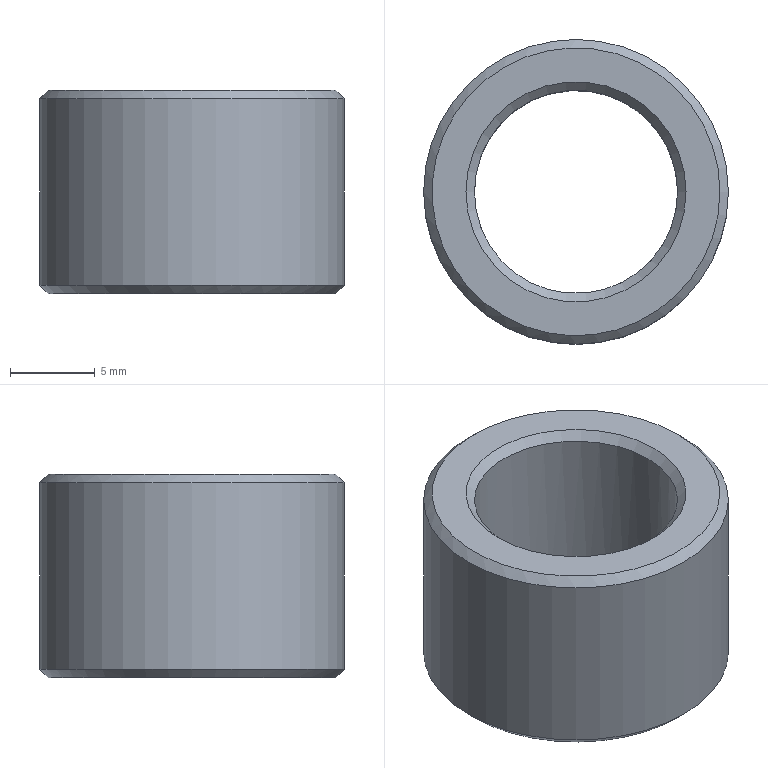Component | NX | BUSHING | 1 solid | 8 faces | box 18 x 18 x 12 mm | volume 1673 mm3 | cone 4 | plane 2 | cylinder 2 | commonest cylinder face diameters 18 x1 12 x1
STEP:
#1=CARTESIAN_POINT('',(0.,0.,0.));
#2=DIRECTION('',(0.,0.,1.));
#3=DIRECTION('',(1.,0.,0.));
#4=AXIS2_PLACEMENT_3D('',#1,#2,#3);
#5=CARTESIAN_POINT('',(17.728,-17.527,-161.719));
#6=VERTEX_POINT('',#5);
#7=CARTESIAN_POINT('',(11.228,-17.527,-161.719));
#8=DIRECTION('',(0.,0.,-1.));
#9=DIRECTION('',(1.,0.,0.));
#10=AXIS2_PLACEMENT_3D('',#7,#8,#9);
#11=CIRCLE('',#10,6.5);
#12=CARTESIAN_POINT('',(11.228,-17.527,-161.719));
#13=DIRECTION('',(0.,0.,1.));
#14=DIRECTION('',(1.,0.,0.));
#15=AXIS2_PLACEMENT_3D('',#12,#13,#14);
#16=PLANE('',#15);
#17=CARTESIAN_POINT('',(6.5,0.));
#18=CARTESIAN_POINT('',(6.5,-11.258));
#19=CARTESIAN_POINT('',(-3.25,-5.629));
#20=CARTESIAN_POINT('',(-13.,-0.));
#21=CARTESIAN_POINT('',(-3.25,5.629));
#22=CARTESIAN_POINT('',(6.5,11.258));
#23=CARTESIAN_POINT('',(6.5,0.));
#24=(BOUNDED_CURVE()B_SPLINE_CURVE(2,(#17,#18,#19,#20,#21,#22,#23),.UNSPECIFIED.,.T.,.F.)B_SPLINE_CURVE_WITH_KNOTS((1,2,2,2,2,1),(-2.094,0.,2.094,4.189,6.283,8.378),.UNSPECIFIED.)CURVE()GEOMETRIC_REPRESENTATION_ITEM()RATIONAL_B_SPLINE_CURVE((1.,0.5,1.,0.5,1.,0.5,1.))REPRESENTATION_ITEM(''));
#25=(GEOMETRIC_REPRESENTATION_CONTEXT(2)PARAMETRIC_REPRESENTATION_CONTEXT()REPRESENTATION_CONTEXT('',''));
#26=DEFINITIONAL_REPRESENTATION('',(#24),#25);
#27=PCURVE('',#16,#26);
#28=CARTESIAN_POINT('',(11.228,-17.527,-161.719));
#29=DIRECTION('',(0.,0.,1.));
#30=DIRECTION('',(1.,0.,0.));
#31=AXIS2_PLACEMENT_3D('',#28,#29,#30);
#32=CONICAL_SURFACE('',#31,6.5,0.7854);
#33=CARTESIAN_POINT('',(6.283,0.));
#34=DIRECTION('',(-1.,0.));
#35=VECTOR('',#34,1.);
#36=LINE('',#33,#35);
#37=(GEOMETRIC_REPRESENTATION_CONTEXT(2)PARAMETRIC_REPRESENTATION_CONTEXT()REPRESENTATION_CONTEXT('',''));
#38=DEFINITIONAL_REPRESENTATION('',(#36),#37);
#39=PCURVE('',#32,#38);
#40=SURFACE_CURVE('',#11,(#27,#39),.PCURVE_S1.);
#41=EDGE_CURVE('',#6,#6,#40,.T.);
#42=ORIENTED_EDGE('',*,*,#41,.T.);
#43=EDGE_LOOP('',(#42));
#44=FACE_BOUND('',#43,.T.);
#45=CARTESIAN_POINT('',(19.728,-17.527,-161.719));
#46=VERTEX_POINT('',#45);
#47=CARTESIAN_POINT('',(11.228,-17.527,-161.719));
#48=DIRECTION('',(0.,0.,1.));
#49=DIRECTION('',(1.,0.,0.));
#50=AXIS2_PLACEMENT_3D('',#47,#48,#49);
#51=CIRCLE('',#50,8.5);
#52=CARTESIAN_POINT('',(0.,0.));
#53=DIRECTION('',(1.,0.));
#54=AXIS2_PLACEMENT_2D('',#52,#53);
#55=CIRCLE('',#54,8.5);
#56=(GEOMETRIC_REPRESENTATION_CONTEXT(2)PARAMETRIC_REPRESENTATION_CONTEXT()REPRESENTATION_CONTEXT('',''));
#57=DEFINITIONAL_REPRESENTATION('',(#55),#56);
#58=PCURVE('',#16,#57);
#59=CARTESIAN_POINT('',(11.228,-17.527,-162.219));
#60=DIRECTION('',(0.,0.,-1.));
#61=DIRECTION('',(-1.,0.,0.));
#62=AXIS2_PLACEMENT_3D('',#59,#60,#61);
#63=CONICAL_SURFACE('',#62,9.,0.7854);
#64=CARTESIAN_POINT('',(9.425,-0.5));
#65=DIRECTION('',(-1.,0.));
#66=VECTOR('',#65,1.);
#67=LINE('',#64,#66);
#68=(GEOMETRIC_REPRESENTATION_CONTEXT(2)PARAMETRIC_REPRESENTATION_CONTEXT()REPRESENTATION_CONTEXT('',''));
#69=DEFINITIONAL_REPRESENTATION('',(#67),#68);
#70=PCURVE('',#63,#69);
#71=SURFACE_CURVE('',#51,(#58,#70),.PCURVE_S1.);
#72=EDGE_CURVE('',#46,#46,#71,.T.);
#73=ORIENTED_EDGE('',*,*,#72,.T.);
#74=EDGE_LOOP('',(#73));
#75=FACE_BOUND('',#74,.T.);
#76=ADVANCED_FACE('',(#44,#75),#16,.T.);
#77=CARTESIAN_POINT('',(4.728,-17.527,-173.719));
#78=VERTEX_POINT('',#77);
#79=CARTESIAN_POINT('',(11.228,-17.527,-173.719));
#80=DIRECTION('',(0.,0.,1.));
#81=DIRECTION('',(-1.,0.,0.));
#82=AXIS2_PLACEMENT_3D('',#79,#80,#81);
#83=CIRCLE('',#82,6.5);
#84=CARTESIAN_POINT('',(11.228,-17.527,-173.719));
#85=DIRECTION('',(0.,0.,-1.));
#86=DIRECTION('',(-1.,0.,0.));
#87=AXIS2_PLACEMENT_3D('',#84,#85,#86);
#88=PLANE('',#87);
#89=CARTESIAN_POINT('',(6.5,0.));
#90=CARTESIAN_POINT('',(6.5,-11.258));
#91=CARTESIAN_POINT('',(-3.25,-5.629));
#92=CARTESIAN_POINT('',(-13.,-0.));
#93=CARTESIAN_POINT('',(-3.25,5.629));
#94=CARTESIAN_POINT('',(6.5,11.258));
#95=CARTESIAN_POINT('',(6.5,0.));
#96=(BOUNDED_CURVE()B_SPLINE_CURVE(2,(#89,#90,#91,#92,#93,#94,#95),.UNSPECIFIED.,.T.,.F.)B_SPLINE_CURVE_WITH_KNOTS((1,2,2,2,2,1),(-2.094,0.,2.094,4.189,6.283,8.378),.UNSPECIFIED.)CURVE()GEOMETRIC_REPRESENTATION_ITEM()RATIONAL_B_SPLINE_CURVE((1.,0.5,1.,0.5,1.,0.5,1.))REPRESENTATION_ITEM(''));
#97=(GEOMETRIC_REPRESENTATION_CONTEXT(2)PARAMETRIC_REPRESENTATION_CONTEXT()REPRESENTATION_CONTEXT('',''));
#98=DEFINITIONAL_REPRESENTATION('',(#96),#97);
#99=PCURVE('',#88,#98);
#100=CARTESIAN_POINT('',(11.228,-17.527,-173.219));
#101=DIRECTION('',(0.,0.,-1.));
#102=DIRECTION('',(-1.,0.,0.));
#103=AXIS2_PLACEMENT_3D('',#100,#101,#102);
#104=CONICAL_SURFACE('',#103,6.,0.7854);
#105=CARTESIAN_POINT('',(6.283,0.5));
#106=DIRECTION('',(-1.,0.));
#107=VECTOR('',#106,1.);
#108=LINE('',#105,#107);
#109=(GEOMETRIC_REPRESENTATION_CONTEXT(2)PARAMETRIC_REPRESENTATION_CONTEXT()REPRESENTATION_CONTEXT('',''));
#110=DEFINITIONAL_REPRESENTATION('',(#108),#109);
#111=PCURVE('',#104,#110);
#112=SURFACE_CURVE('',#83,(#99,#111),.PCURVE_S1.);
#113=EDGE_CURVE('',#78,#78,#112,.T.);
#114=ORIENTED_EDGE('',*,*,#113,.T.);
#115=EDGE_LOOP('',(#114));
#116=FACE_BOUND('',#115,.T.);
#117=CARTESIAN_POINT('',(2.728,-17.527,-173.719));
#118=VERTEX_POINT('',#117);
#119=CARTESIAN_POINT('',(11.228,-17.527,-173.719));
#120=DIRECTION('',(0.,0.,-1.));
#121=DIRECTION('',(-1.,0.,0.));
#122=AXIS2_PLACEMENT_3D('',#119,#120,#121);
#123=CIRCLE('',#122,8.5);
#124=CARTESIAN_POINT('',(0.,0.));
#125=DIRECTION('',(1.,0.));
#126=AXIS2_PLACEMENT_2D('',#124,#125);
#127=CIRCLE('',#126,8.5);
#128=(GEOMETRIC_REPRESENTATION_CONTEXT(2)PARAMETRIC_REPRESENTATION_CONTEXT()REPRESENTATION_CONTEXT('',''));
#129=DEFINITIONAL_REPRESENTATION('',(#127),#128);
#130=PCURVE('',#88,#129);
#131=CARTESIAN_POINT('',(11.228,-17.527,-173.219));
#132=DIRECTION('',(0.,0.,1.));
#133=DIRECTION('',(1.,0.,0.));
#134=AXIS2_PLACEMENT_3D('',#131,#132,#133);
#135=CONICAL_SURFACE('',#134,9.,0.7854);
#136=CARTESIAN_POINT('',(9.425,-0.5));
#137=DIRECTION('',(-1.,0.));
#138=VECTOR('',#137,1.);
#139=LINE('',#136,#138);
#140=(GEOMETRIC_REPRESENTATION_CONTEXT(2)PARAMETRIC_REPRESENTATION_CONTEXT()REPRESENTATION_CONTEXT('',''));
#141=DEFINITIONAL_REPRESENTATION('',(#139),#140);
#142=PCURVE('',#135,#141);
#143=SURFACE_CURVE('',#123,(#130,#142),.PCURVE_S1.);
#144=EDGE_CURVE('',#118,#118,#143,.T.);
#145=ORIENTED_EDGE('',*,*,#144,.T.);
#146=EDGE_LOOP('',(#145));
#147=FACE_BOUND('',#146,.T.);
#148=ADVANCED_FACE('',(#116,#147),#88,.T.);
#149=CARTESIAN_POINT('',(2.228,-17.527,-173.219));
#150=VERTEX_POINT('',#149);
#151=CARTESIAN_POINT('',(20.228,-17.527,-173.219));
#152=VERTEX_POINT('',#151);
#153=CARTESIAN_POINT('',(11.228,-17.527,-173.219));
#154=DIRECTION('',(0.,0.,1.));
#155=DIRECTION('',(-1.,0.,0.));
#156=AXIS2_PLACEMENT_3D('',#153,#154,#155);
#157=CIRCLE('',#156,9.);
#158=CARTESIAN_POINT('',(11.228,-17.527,-173.719));
#159=DIRECTION('',(0.,0.,1.));
#160=DIRECTION('',(1.,0.,0.));
#161=AXIS2_PLACEMENT_3D('',#158,#159,#160);
#162=CYLINDRICAL_SURFACE('',#161,9.);
#163=CARTESIAN_POINT('',(3.142,0.5));
#164=DIRECTION('',(1.,0.));
#165=VECTOR('',#164,1.);
#166=LINE('',#163,#165);
#167=(GEOMETRIC_REPRESENTATION_CONTEXT(2)PARAMETRIC_REPRESENTATION_CONTEXT()REPRESENTATION_CONTEXT('',''));
#168=DEFINITIONAL_REPRESENTATION('',(#166),#167);
#169=PCURVE('',#162,#168);
#170=CARTESIAN_POINT('',(3.142,0.));
#171=DIRECTION('',(1.,0.));
#172=VECTOR('',#171,1.);
#173=LINE('',#170,#172);
#174=(GEOMETRIC_REPRESENTATION_CONTEXT(2)PARAMETRIC_REPRESENTATION_CONTEXT()REPRESENTATION_CONTEXT('',''));
#175=DEFINITIONAL_REPRESENTATION('',(#173),#174);
#176=PCURVE('',#135,#175);
#177=SURFACE_CURVE('',#157,(#169,#176),.PCURVE_S1.);
#178=EDGE_CURVE('',#150,#152,#177,.T.);
#179=ORIENTED_EDGE('',*,*,#178,.T.);
#180=CARTESIAN_POINT('',(20.228,-17.527,-162.219));
#181=VERTEX_POINT('',#180);
#182=CARTESIAN_POINT('',(20.228,-17.527,-173.219));
#183=CARTESIAN_POINT('',(20.228,-17.527,-162.219));
#184=B_SPLINE_CURVE_WITH_KNOTS('',1,(#182,#183),.UNSPECIFIED.,.F.,.F.,(2,2),(0.5,11.5),.PIECEWISE_BEZIER_KNOTS.);
#185=CARTESIAN_POINT('',(6.283,0.));
#186=DIRECTION('',(0.,1.));
#187=VECTOR('',#186,1.);
#188=LINE('',#185,#187);
#189=(GEOMETRIC_REPRESENTATION_CONTEXT(2)PARAMETRIC_REPRESENTATION_CONTEXT()REPRESENTATION_CONTEXT('',''));
#190=DEFINITIONAL_REPRESENTATION('',(#188),#189);
#191=PCURVE('',#162,#190);
#192=CARTESIAN_POINT('',(0.,0.));
#193=DIRECTION('',(0.,1.));
#194=VECTOR('',#193,1.);
#195=LINE('',#192,#194);
#196=(GEOMETRIC_REPRESENTATION_CONTEXT(2)PARAMETRIC_REPRESENTATION_CONTEXT()REPRESENTATION_CONTEXT('',''));
#197=DEFINITIONAL_REPRESENTATION('',(#195),#196);
#198=PCURVE('',#162,#197);
#199=SEAM_CURVE('',#184,(#191,#198),.PCURVE_S1.);
#200=EDGE_CURVE('',#152,#181,#199,.T.);
#201=ORIENTED_EDGE('',*,*,#200,.T.);
#202=CARTESIAN_POINT('',(11.228,-17.527,-162.219));
#203=DIRECTION('',(0.,0.,-1.));
#204=DIRECTION('',(1.,0.,0.));
#205=AXIS2_PLACEMENT_3D('',#202,#203,#204);
#206=CIRCLE('',#205,9.);
#207=CARTESIAN_POINT('',(6.283,11.5));
#208=DIRECTION('',(-1.,0.));
#209=VECTOR('',#208,1.);
#210=LINE('',#207,#209);
#211=(GEOMETRIC_REPRESENTATION_CONTEXT(2)PARAMETRIC_REPRESENTATION_CONTEXT()REPRESENTATION_CONTEXT('',''));
#212=DEFINITIONAL_REPRESENTATION('',(#210),#211);
#213=PCURVE('',#162,#212);
#214=CARTESIAN_POINT('',(3.142,0.));
#215=DIRECTION('',(1.,0.));
#216=VECTOR('',#215,1.);
#217=LINE('',#214,#216);
#218=(GEOMETRIC_REPRESENTATION_CONTEXT(2)PARAMETRIC_REPRESENTATION_CONTEXT()REPRESENTATION_CONTEXT('',''));
#219=DEFINITIONAL_REPRESENTATION('',(#217),#218);
#220=PCURVE('',#63,#219);
#221=SURFACE_CURVE('',#206,(#213,#220),.PCURVE_S1.);
#222=EDGE_CURVE('',#181,#181,#221,.T.);
#223=ORIENTED_EDGE('',*,*,#222,.T.);
#224=ORIENTED_EDGE('',*,*,#200,.F.);
#225=CARTESIAN_POINT('',(11.228,-17.527,-173.219));
#226=DIRECTION('',(0.,0.,1.));
#227=DIRECTION('',(-1.,0.,0.));
#228=AXIS2_PLACEMENT_3D('',#225,#226,#227);
#229=CIRCLE('',#228,9.);
#230=CARTESIAN_POINT('',(-3.142,0.5));
#231=DIRECTION('',(1.,0.));
#232=VECTOR('',#231,1.);
#233=LINE('',#230,#232);
#234=(GEOMETRIC_REPRESENTATION_CONTEXT(2)PARAMETRIC_REPRESENTATION_CONTEXT()REPRESENTATION_CONTEXT('',''));
#235=DEFINITIONAL_REPRESENTATION('',(#233),#234);
#236=PCURVE('',#162,#235);
#237=CARTESIAN_POINT('',(3.142,0.));
#238=DIRECTION('',(1.,0.));
#239=VECTOR('',#238,1.);
#240=LINE('',#237,#239);
#241=(GEOMETRIC_REPRESENTATION_CONTEXT(2)PARAMETRIC_REPRESENTATION_CONTEXT()REPRESENTATION_CONTEXT('',''));
#242=DEFINITIONAL_REPRESENTATION('',(#240),#241);
#243=PCURVE('',#135,#242);
#244=SURFACE_CURVE('',#229,(#236,#243),.PCURVE_S1.);
#245=EDGE_CURVE('',#152,#150,#244,.T.);
#246=ORIENTED_EDGE('',*,*,#245,.T.);
#247=EDGE_LOOP('',(#179,#201,#223,#224,#246));
#248=FACE_BOUND('',#247,.T.);
#249=ADVANCED_FACE('',(#248),#162,.T.);
#250=CARTESIAN_POINT('',(5.228,-17.527,-173.219));
#251=VERTEX_POINT('',#250);
#252=CARTESIAN_POINT('',(11.228,-17.527,-173.219));
#253=DIRECTION('',(0.,0.,-1.));
#254=DIRECTION('',(-1.,0.,0.));
#255=AXIS2_PLACEMENT_3D('',#252,#253,#254);
#256=CIRCLE('',#255,6.);
#257=CARTESIAN_POINT('',(11.228,-17.527,-161.719));
#258=DIRECTION('',(0.,0.,-1.));
#259=DIRECTION('',(-1.,0.,0.));
#260=AXIS2_PLACEMENT_3D('',#257,#258,#259);
#261=CYLINDRICAL_SURFACE('',#260,6.);
#262=CARTESIAN_POINT('',(0.,11.5));
#263=DIRECTION('',(1.,0.));
#264=VECTOR('',#263,1.);
#265=LINE('',#262,#264);
#266=(GEOMETRIC_REPRESENTATION_CONTEXT(2)PARAMETRIC_REPRESENTATION_CONTEXT()REPRESENTATION_CONTEXT('',''));
#267=DEFINITIONAL_REPRESENTATION('',(#265),#266);
#268=PCURVE('',#261,#267);
#269=CARTESIAN_POINT('',(0.,0.));
#270=DIRECTION('',(1.,0.));
#271=VECTOR('',#270,1.);
#272=LINE('',#269,#271);
#273=(GEOMETRIC_REPRESENTATION_CONTEXT(2)PARAMETRIC_REPRESENTATION_CONTEXT()REPRESENTATION_CONTEXT('',''));
#274=DEFINITIONAL_REPRESENTATION('',(#272),#273);
#275=PCURVE('',#104,#274);
#276=SURFACE_CURVE('',#256,(#268,#275),.PCURVE_S1.);
#277=EDGE_CURVE('',#251,#251,#276,.T.);
#278=ORIENTED_EDGE('',*,*,#277,.F.);
#279=CARTESIAN_POINT('',(5.228,-17.527,-162.219));
#280=VERTEX_POINT('',#279);
#281=CARTESIAN_POINT('',(5.228,-17.527,-162.219));
#282=CARTESIAN_POINT('',(5.228,-17.527,-173.219));
#283=B_SPLINE_CURVE_WITH_KNOTS('',1,(#281,#282),.UNSPECIFIED.,.F.,.F.,(2,2),(0.5,11.5),.PIECEWISE_BEZIER_KNOTS.);
#284=CARTESIAN_POINT('',(0.,0.));
#285=DIRECTION('',(0.,1.));
#286=VECTOR('',#285,1.);
#287=LINE('',#284,#286);
#288=(GEOMETRIC_REPRESENTATION_CONTEXT(2)PARAMETRIC_REPRESENTATION_CONTEXT()REPRESENTATION_CONTEXT('',''));
#289=DEFINITIONAL_REPRESENTATION('',(#287),#288);
#290=PCURVE('',#261,#289);
#291=CARTESIAN_POINT('',(6.283,0.));
#292=DIRECTION('',(0.,1.));
#293=VECTOR('',#292,1.);
#294=LINE('',#291,#293);
#295=(GEOMETRIC_REPRESENTATION_CONTEXT(2)PARAMETRIC_REPRESENTATION_CONTEXT()REPRESENTATION_CONTEXT('',''));
#296=DEFINITIONAL_REPRESENTATION('',(#294),#295);
#297=PCURVE('',#261,#296);
#298=SEAM_CURVE('',#283,(#290,#297),.PCURVE_S1.);
#299=EDGE_CURVE('',#280,#251,#298,.T.);
#300=ORIENTED_EDGE('',*,*,#299,.F.);
#301=CARTESIAN_POINT('',(17.228,-17.527,-162.219));
#302=VERTEX_POINT('',#301);
#303=CARTESIAN_POINT('',(11.228,-17.527,-162.219));
#304=DIRECTION('',(0.,0.,1.));
#305=DIRECTION('',(1.,0.,0.));
#306=AXIS2_PLACEMENT_3D('',#303,#304,#305);
#307=CIRCLE('',#306,6.);
#308=CARTESIAN_POINT('',(3.142,0.5));
#309=DIRECTION('',(-1.,0.));
#310=VECTOR('',#309,1.);
#311=LINE('',#308,#310);
#312=(GEOMETRIC_REPRESENTATION_CONTEXT(2)PARAMETRIC_REPRESENTATION_CONTEXT()REPRESENTATION_CONTEXT('',''));
#313=DEFINITIONAL_REPRESENTATION('',(#311),#312);
#314=PCURVE('',#261,#313);
#315=CARTESIAN_POINT('',(0.,-0.5));
#316=DIRECTION('',(1.,0.));
#317=VECTOR('',#316,1.);
#318=LINE('',#315,#317);
#319=(GEOMETRIC_REPRESENTATION_CONTEXT(2)PARAMETRIC_REPRESENTATION_CONTEXT()REPRESENTATION_CONTEXT('',''));
#320=DEFINITIONAL_REPRESENTATION('',(#318),#319);
#321=PCURVE('',#32,#320);
#322=SURFACE_CURVE('',#307,(#314,#321),.PCURVE_S1.);
#323=EDGE_CURVE('',#302,#280,#322,.T.);
#324=ORIENTED_EDGE('',*,*,#323,.F.);
#325=CARTESIAN_POINT('',(11.228,-17.527,-162.219));
#326=DIRECTION('',(0.,0.,1.));
#327=DIRECTION('',(1.,0.,0.));
#328=AXIS2_PLACEMENT_3D('',#325,#326,#327);
#329=CIRCLE('',#328,6.);
#330=CARTESIAN_POINT('',(9.425,0.5));
#331=DIRECTION('',(-1.,0.));
#332=VECTOR('',#331,1.);
#333=LINE('',#330,#332);
#334=(GEOMETRIC_REPRESENTATION_CONTEXT(2)PARAMETRIC_REPRESENTATION_CONTEXT()REPRESENTATION_CONTEXT('',''));
#335=DEFINITIONAL_REPRESENTATION('',(#333),#334);
#336=PCURVE('',#261,#335);
#337=CARTESIAN_POINT('',(0.,-0.5));
#338=DIRECTION('',(1.,0.));
#339=VECTOR('',#338,1.);
#340=LINE('',#337,#339);
#341=(GEOMETRIC_REPRESENTATION_CONTEXT(2)PARAMETRIC_REPRESENTATION_CONTEXT()REPRESENTATION_CONTEXT('',''));
#342=DEFINITIONAL_REPRESENTATION('',(#340),#341);
#343=PCURVE('',#32,#342);
#344=SURFACE_CURVE('',#329,(#336,#343),.PCURVE_S1.);
#345=EDGE_CURVE('',#280,#302,#344,.T.);
#346=ORIENTED_EDGE('',*,*,#345,.F.);
#347=ORIENTED_EDGE('',*,*,#299,.T.);
#348=EDGE_LOOP('',(#278,#300,#324,#346,#347));
#349=FACE_BOUND('',#348,.F.);
#350=ADVANCED_FACE('',(#349),#261,.F.);
#351=ORIENTED_EDGE('',*,*,#113,.T.);
#352=CARTESIAN_POINT('',(5.228,-17.527,-173.219));
#353=CARTESIAN_POINT('',(4.728,-17.527,-173.719));
#354=B_SPLINE_CURVE_WITH_KNOTS('',1,(#352,#353),.UNSPECIFIED.,.F.,.F.,(2,2),(0.,0.7071),.PIECEWISE_BEZIER_KNOTS.);
#355=CARTESIAN_POINT('',(0.,0.));
#356=DIRECTION('',(0.,1.));
#357=VECTOR('',#356,1.);
#358=LINE('',#355,#357);
#359=(GEOMETRIC_REPRESENTATION_CONTEXT(2)PARAMETRIC_REPRESENTATION_CONTEXT()REPRESENTATION_CONTEXT('',''));
#360=DEFINITIONAL_REPRESENTATION('',(#358),#359);
#361=PCURVE('',#104,#360);
#362=CARTESIAN_POINT('',(6.283,0.));
#363=DIRECTION('',(0.,1.));
#364=VECTOR('',#363,1.);
#365=LINE('',#362,#364);
#366=(GEOMETRIC_REPRESENTATION_CONTEXT(2)PARAMETRIC_REPRESENTATION_CONTEXT()REPRESENTATION_CONTEXT('',''));
#367=DEFINITIONAL_REPRESENTATION('',(#365),#366);
#368=PCURVE('',#104,#367);
#369=SEAM_CURVE('',#354,(#361,#368),.PCURVE_S1.);
#370=EDGE_CURVE('',#251,#78,#369,.T.);
#371=ORIENTED_EDGE('',*,*,#370,.F.);
#372=ORIENTED_EDGE('',*,*,#277,.T.);
#373=ORIENTED_EDGE('',*,*,#370,.T.);
#374=EDGE_LOOP('',(#351,#371,#372,#373));
#375=FACE_BOUND('',#374,.F.);
#376=ADVANCED_FACE('',(#375),#104,.F.);
#377=ORIENTED_EDGE('',*,*,#144,.F.);
#378=CARTESIAN_POINT('',(2.728,-17.527,-173.719));
#379=CARTESIAN_POINT('',(2.228,-17.527,-173.219));
#380=B_SPLINE_CURVE_WITH_KNOTS('',1,(#378,#379),.UNSPECIFIED.,.F.,.F.,(2,2),(-0.7071,0.),.PIECEWISE_BEZIER_KNOTS.);
#381=CARTESIAN_POINT('',(9.425,0.));
#382=DIRECTION('',(0.,1.));
#383=VECTOR('',#382,1.);
#384=LINE('',#381,#383);
#385=(GEOMETRIC_REPRESENTATION_CONTEXT(2)PARAMETRIC_REPRESENTATION_CONTEXT()REPRESENTATION_CONTEXT('',''));
#386=DEFINITIONAL_REPRESENTATION('',(#384),#385);
#387=PCURVE('',#135,#386);
#388=CARTESIAN_POINT('',(3.142,0.));
#389=DIRECTION('',(0.,1.));
#390=VECTOR('',#389,1.);
#391=LINE('',#388,#390);
#392=(GEOMETRIC_REPRESENTATION_CONTEXT(2)PARAMETRIC_REPRESENTATION_CONTEXT()REPRESENTATION_CONTEXT('',''));
#393=DEFINITIONAL_REPRESENTATION('',(#391),#392);
#394=PCURVE('',#135,#393);
#395=SEAM_CURVE('',#380,(#387,#394),.PCURVE_S1.);
#396=EDGE_CURVE('',#118,#150,#395,.T.);
#397=ORIENTED_EDGE('',*,*,#396,.T.);
#398=ORIENTED_EDGE('',*,*,#245,.F.);
#399=ORIENTED_EDGE('',*,*,#178,.F.);
#400=ORIENTED_EDGE('',*,*,#396,.F.);
#401=EDGE_LOOP('',(#377,#397,#398,#399,#400));
#402=FACE_BOUND('',#401,.T.);
#403=ADVANCED_FACE('',(#402),#135,.T.);
#404=ORIENTED_EDGE('',*,*,#345,.T.);
#405=CARTESIAN_POINT('',(17.228,-17.527,-162.219));
#406=CARTESIAN_POINT('',(17.728,-17.527,-161.719));
#407=B_SPLINE_CURVE_WITH_KNOTS('',1,(#405,#406),.UNSPECIFIED.,.F.,.F.,(2,2),(-0.7071,0.),.PIECEWISE_BEZIER_KNOTS.);
#408=CARTESIAN_POINT('',(6.283,0.));
#409=DIRECTION('',(0.,1.));
#410=VECTOR('',#409,1.);
#411=LINE('',#408,#410);
#412=(GEOMETRIC_REPRESENTATION_CONTEXT(2)PARAMETRIC_REPRESENTATION_CONTEXT()REPRESENTATION_CONTEXT('',''));
#413=DEFINITIONAL_REPRESENTATION('',(#411),#412);
#414=PCURVE('',#32,#413);
#415=CARTESIAN_POINT('',(0.,0.));
#416=DIRECTION('',(0.,1.));
#417=VECTOR('',#416,1.);
#418=LINE('',#415,#417);
#419=(GEOMETRIC_REPRESENTATION_CONTEXT(2)PARAMETRIC_REPRESENTATION_CONTEXT()REPRESENTATION_CONTEXT('',''));
#420=DEFINITIONAL_REPRESENTATION('',(#418),#419);
#421=PCURVE('',#32,#420);
#422=SEAM_CURVE('',#407,(#414,#421),.PCURVE_S1.);
#423=EDGE_CURVE('',#302,#6,#422,.T.);
#424=ORIENTED_EDGE('',*,*,#423,.T.);
#425=ORIENTED_EDGE('',*,*,#41,.T.);
#426=ORIENTED_EDGE('',*,*,#423,.F.);
#427=ORIENTED_EDGE('',*,*,#323,.T.);
#428=EDGE_LOOP('',(#404,#424,#425,#426,#427));
#429=FACE_BOUND('',#428,.F.);
#430=ADVANCED_FACE('',(#429),#32,.F.);
#431=ORIENTED_EDGE('',*,*,#72,.F.);
#432=CARTESIAN_POINT('',(19.728,-17.527,-161.719));
#433=CARTESIAN_POINT('',(20.228,-17.527,-162.219));
#434=B_SPLINE_CURVE_WITH_KNOTS('',1,(#432,#433),.UNSPECIFIED.,.F.,.F.,(2,2),(-0.7071,0.),.PIECEWISE_BEZIER_KNOTS.);
#435=CARTESIAN_POINT('',(9.425,0.));
#436=DIRECTION('',(0.,1.));
#437=VECTOR('',#436,1.);
#438=LINE('',#435,#437);
#439=(GEOMETRIC_REPRESENTATION_CONTEXT(2)PARAMETRIC_REPRESENTATION_CONTEXT()REPRESENTATION_CONTEXT('',''));
#440=DEFINITIONAL_REPRESENTATION('',(#438),#439);
#441=PCURVE('',#63,#440);
#442=CARTESIAN_POINT('',(3.142,0.));
#443=DIRECTION('',(0.,1.));
#444=VECTOR('',#443,1.);
#445=LINE('',#442,#444);
#446=(GEOMETRIC_REPRESENTATION_CONTEXT(2)PARAMETRIC_REPRESENTATION_CONTEXT()REPRESENTATION_CONTEXT('',''));
#447=DEFINITIONAL_REPRESENTATION('',(#445),#446);
#448=PCURVE('',#63,#447);
#449=SEAM_CURVE('',#434,(#441,#448),.PCURVE_S1.);
#450=EDGE_CURVE('',#46,#181,#449,.T.);
#451=ORIENTED_EDGE('',*,*,#450,.T.);
#452=ORIENTED_EDGE('',*,*,#222,.F.);
#453=ORIENTED_EDGE('',*,*,#450,.F.);
#454=EDGE_LOOP('',(#431,#451,#452,#453));
#455=FACE_BOUND('',#454,.T.);
#456=ADVANCED_FACE('',(#455),#63,.T.);
#457=CLOSED_SHELL('',(#76,#148,#249,#350,#376,#403,#430,#456));
#458=MANIFOLD_SOLID_BREP('',#457);
#459=(LENGTH_UNIT()NAMED_UNIT(*)SI_UNIT(.MILLI.,.METRE.));
#460=UNCERTAINTY_MEASURE_WITH_UNIT(LENGTH_MEASURE(0.00001),#459,'','');
#461=(NAMED_UNIT(*)PLANE_ANGLE_UNIT()SI_UNIT($,.RADIAN.));
#462=(NAMED_UNIT(*)SI_UNIT($,.STERADIAN.)SOLID_ANGLE_UNIT());
#463=(GEOMETRIC_REPRESENTATION_CONTEXT(3)GLOBAL_UNCERTAINTY_ASSIGNED_CONTEXT((#460))GLOBAL_UNIT_ASSIGNED_CONTEXT((#459,#461,#462))REPRESENTATION_CONTEXT('',''));
#464=ADVANCED_BREP_SHAPE_REPRESENTATION('',(#4,#458),#463);